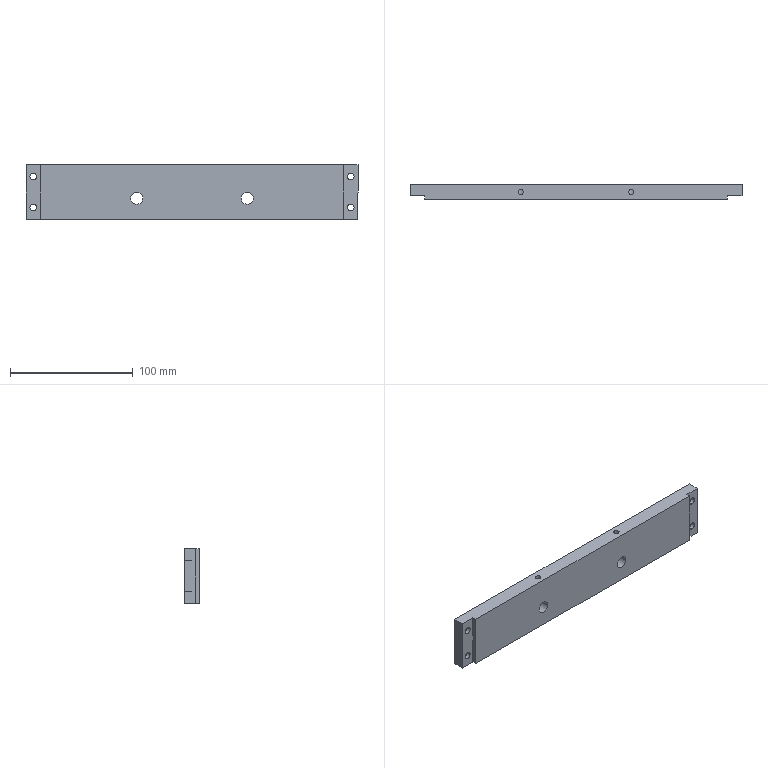Component | SolidWorks | STB-08-044-1 | 1 solid | 50 faces | box 270 x 12 x 44 mm | volume 134486 mm3 | cylinder 30 | plane 14 | cone 6 | commonest cylinder face diameters 10 x12 5.5 x8 3.3 x6 4.2 x4
build123d program:
from build123d import *

# Parameters (mm, degrees)
SKETCH1_W                                            = 44
SKETCH1_H                                            = 270
EXTRUDE1_DEPTH                                       = 6
CUT_EXTRUDE1_REACH                                   = 144.116
SKETCH2_W                                            = 12
SKETCH2_H                                            = 3
HOLE_SIZE_ACCORDING_TO_HEX_SOCKET_HEAD_C_D           = 5.5
HOLE_SIZE_ACCORDING_TO_HEX_SOCKET_HEAD_C_CBORE_D     = 10
HOLE_SIZE_ACCORDING_TO_HEX_SOCKET_HEAD_C_CBORE_DEPTH = 5.7
M4_TAPPED_HOLE1_D                                    = 3.3
M4_TAPPED_HOLE1_DEPTH                                = 11.5
M4_TAPPED_HOLE1_TIP                                  = 0.9914
CUT_EXTRUDE2_REACH                                   = 139.306
SKETCH10_R                                           = 5
M5_TAPPED_HOLE1_REACH                                = 144.116
M5_TAPPED_HOLE1_BORE_R                               = 2.1


with BuildPart() as part:
    # Sketch1 → Extrude1 (new, symmetric)
    with BuildSketch(Plane(origin=(0, 0, 0), x_dir=(1, 0, 0), z_dir=(0, 1, 0))):
        Rectangle(SKETCH1_W, SKETCH1_H)
    extrude(amount=EXTRUDE1_DEPTH, both=True)

    # Sketch2 → Cut-Extrude1 (cut, up to next)
    with BuildSketch(Plane(origin=(22, 0, 0), x_dir=(0, 0, -1), z_dir=(1, 0, 0)), mode=Mode.PRIVATE) as cut_extrude1_sk1:
        with Locations((-129, -4.5)):
            Rectangle(SKETCH2_W, SKETCH2_H)
    cut_extrude1_tool1 = extrude(cut_extrude1_sk1.sketch, amount=-CUT_EXTRUDE1_REACH, mode=Mode.PRIVATE) & part.part
    cut_extrude1 = cut_extrude1_tool1.solids().sort_by_distance((22, -4.5, 129))[0]
    add(cut_extrude1, mode=Mode.SUBTRACT)

    # Mirror1: Cut-Extrude1 across plane
    add(cut_extrude1.mirror(Plane.XY), mode=Mode.SUBTRACT)

    # Hole Size according to Hex Socket Head C (through all)
    with Locations(Plane(origin=(0, 6, 0), x_dir=(-1, 0, 0), z_dir=(0, 1, 0))):
        with Locations((12.5, 129), (-12.5, 129)):
            hole_size_according_to_hex_socket_head_c = CounterBoreHole(HOLE_SIZE_ACCORDING_TO_HEX_SOCKET_HEAD_C_D / 2, HOLE_SIZE_ACCORDING_TO_HEX_SOCKET_HEAD_C_CBORE_D / 2, HOLE_SIZE_ACCORDING_TO_HEX_SOCKET_HEAD_C_CBORE_DEPTH)

    # Mirror2: Hole Size according to Hex Socket Head C across plane
    add(hole_size_according_to_hex_socket_head_c.mirror(Plane.XY), mode=Mode.SUBTRACT)

    # M4 Tapped Hole1
    with Locations(Plane.ZY.offset(22)):
        with Locations((-90, 0), (0, 0), (90, 0)):
            Hole(M4_TAPPED_HOLE1_D / 2, depth=M4_TAPPED_HOLE1_DEPTH)
            with Locations((0, 0, -(M4_TAPPED_HOLE1_DEPTH + M4_TAPPED_HOLE1_TIP / 2))):  # 118° drill point
                Cone(0, M4_TAPPED_HOLE1_D / 2, M4_TAPPED_HOLE1_TIP, mode=Mode.SUBTRACT)

    # Sketch10 → Cut-Extrude2 (cut, up to next)
    with BuildSketch(Plane(origin=(0, 6, 0), x_dir=(1, 0, 0), z_dir=(0, 1, 0)), mode=Mode.PRIVATE) as cut_extrude2_sk1:
        with Locations(Location((-5, 45, 0), (0, 0, 270))):
            Circle(SKETCH10_R)
    cut_extrude2_tool1 = extrude(cut_extrude2_sk1.sketch, amount=-CUT_EXTRUDE2_REACH, mode=Mode.PRIVATE) & part.part
    # Sketch10 → Cut-Extrude2 (cut, up to next)
    with BuildSketch(Plane(origin=(0, 6, 0), x_dir=(1, 0, 0), z_dir=(0, 1, 0)), mode=Mode.PRIVATE) as cut_extrude2_sk2:
        with Locations(Location((-5, -45, 0), (0, 0, 270))):
            Circle(SKETCH10_R)
    cut_extrude2_tool2 = extrude(cut_extrude2_sk2.sketch, amount=-CUT_EXTRUDE2_REACH, mode=Mode.PRIVATE) & part.part
    add(cut_extrude2_tool1.solids().sort_by_distance((-5, 6, -45))[0], mode=Mode.SUBTRACT)
    add(cut_extrude2_tool2.solids().sort_by_distance((-5, 6, 45))[0], mode=Mode.SUBTRACT)

    # M5 Tapped Hole1 bore → M5 Tapped Hole1 (cut, up to next)
    with BuildSketch(Plane(origin=(22, 0, 0), x_dir=(0, 0, -1), z_dir=(1, 0, 0)), mode=Mode.PRIVATE) as m5_tapped_hole1_sk1:
        with Locations((-45, 0)):
            Circle(M5_TAPPED_HOLE1_BORE_R)
    m5_tapped_hole1_tool1 = extrude(m5_tapped_hole1_sk1.sketch, amount=-M5_TAPPED_HOLE1_REACH, mode=Mode.PRIVATE) & part.part
    # M5 Tapped Hole1 bore → M5 Tapped Hole1 (cut, up to next)
    with BuildSketch(Plane(origin=(22, 0, 0), x_dir=(0, 0, -1), z_dir=(1, 0, 0)), mode=Mode.PRIVATE) as m5_tapped_hole1_sk2:
        with Locations((45, 0)):
            Circle(M5_TAPPED_HOLE1_BORE_R)
    m5_tapped_hole1_tool2 = extrude(m5_tapped_hole1_sk2.sketch, amount=-M5_TAPPED_HOLE1_REACH, mode=Mode.PRIVATE) & part.part
    add(m5_tapped_hole1_tool1.solids().sort_by_distance((22, 0, 45))[0], mode=Mode.SUBTRACT)
    add(m5_tapped_hole1_tool2.solids().sort_by_distance((22, 0, -45))[0], mode=Mode.SUBTRACT)


solid = part.part

# Placed as in the assembly
solid = solid.moved(Location((-104.904, 460.999, -7), (0, -90, 0)))